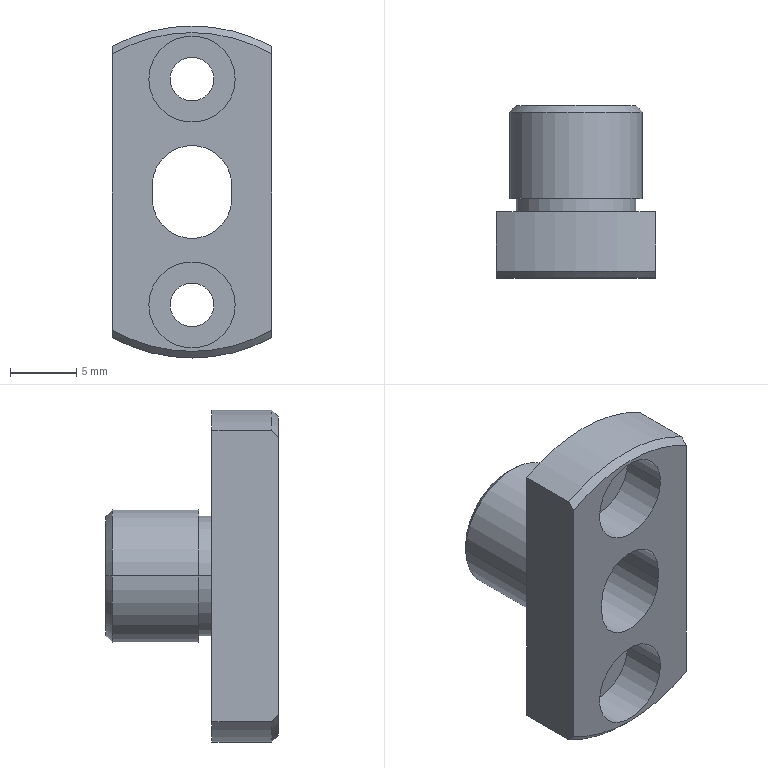Component | SolidWorks | F-JBEH10-P7-W6-L8-1 | 1 solid | 30 faces | box 12 x 13 x 25 mm | volume 1343 mm3 | cylinder 16 | plane 10 | cone 4 | commonest cylinder face diameters 3.3 x4 6.5 x4 9 x2 10 x2 25 x2 6 x2
STEP:
#1=COLOUR_RGB('',0.7922,0.8196,0.9333);
#2=FILL_AREA_STYLE_COLOUR('',#1);
#3=FILL_AREA_STYLE('',(#2));
#4=SURFACE_STYLE_FILL_AREA(#3);
#5=SURFACE_SIDE_STYLE('',(#4));
#6=SURFACE_STYLE_USAGE(.BOTH.,#5);
#7=PRESENTATION_STYLE_ASSIGNMENT((#6));
#8=CARTESIAN_POINT('',(-4.175,-1.116,4.536));
#9=VERTEX_POINT('',#8);
#10=CARTESIAN_POINT('',(-4.305,-1.116,4.536));
#11=VERTEX_POINT('',#10);
#12=CARTESIAN_POINT('',(-4.24,-1.116,4.536));
#13=DIRECTION('',(0.,1.,0.));
#14=DIRECTION('',(1.,0.,0.));
#15=AXIS2_PLACEMENT_3D('',#12,#13,#14);
#16=CIRCLE('',#15,0.06496);
#17=EDGE_CURVE('',#9,#11,#16,.T.);
#18=ORIENTED_EDGE('',*,*,#17,.T.);
#19=CARTESIAN_POINT('',(-4.305,-1.175,4.536));
#20=VERTEX_POINT('',#19);
#21=CARTESIAN_POINT('',(-4.305,-1.116,4.536));
#22=DIRECTION('',(0.,-1.,0.));
#23=VECTOR('',#22,39.37);
#24=LINE('',#21,#23);
#25=EDGE_CURVE('',#11,#20,#24,.T.);
#26=ORIENTED_EDGE('',*,*,#25,.T.);
#27=CARTESIAN_POINT('',(-4.175,-1.175,4.536));
#28=VERTEX_POINT('',#27);
#29=CARTESIAN_POINT('',(-4.24,-1.175,4.536));
#30=DIRECTION('',(0.,1.,0.));
#31=DIRECTION('',(1.,0.,0.));
#32=AXIS2_PLACEMENT_3D('',#29,#30,#31);
#33=CIRCLE('',#32,0.06496);
#34=EDGE_CURVE('',#28,#20,#33,.T.);
#35=ORIENTED_EDGE('',*,*,#34,.F.);
#36=CARTESIAN_POINT('',(-4.175,-1.116,4.536));
#37=DIRECTION('',(0.,-1.,0.));
#38=VECTOR('',#37,39.37);
#39=LINE('',#36,#38);
#40=EDGE_CURVE('',#9,#28,#39,.T.);
#41=ORIENTED_EDGE('',*,*,#40,.F.);
#42=EDGE_LOOP('',(#18,#26,#35,#41));
#43=FACE_OUTER_BOUND('',#42,.T.);
#44=CARTESIAN_POINT('',(-4.24,-1.116,4.536));
#45=DIRECTION('',(0.,-1.,0.));
#46=DIRECTION('',(1.,0.,0.));
#47=AXIS2_PLACEMENT_3D('',#44,#45,#46);
#48=CYLINDRICAL_SURFACE('',#47,0.06496);
#49=ADVANCED_FACE('',(#43),#48,.F.);
#50=CARTESIAN_POINT('',(-4.175,-1.116,5.206));
#51=VERTEX_POINT('',#50);
#52=CARTESIAN_POINT('',(-4.305,-1.116,5.206));
#53=VERTEX_POINT('',#52);
#54=CARTESIAN_POINT('',(-4.24,-1.116,5.206));
#55=DIRECTION('',(0.,1.,0.));
#56=DIRECTION('',(1.,0.,0.));
#57=AXIS2_PLACEMENT_3D('',#54,#55,#56);
#58=CIRCLE('',#57,0.06496);
#59=EDGE_CURVE('',#51,#53,#58,.T.);
#60=ORIENTED_EDGE('',*,*,#59,.T.);
#61=CARTESIAN_POINT('',(-4.305,-1.175,5.206));
#62=VERTEX_POINT('',#61);
#63=CARTESIAN_POINT('',(-4.305,-1.116,5.206));
#64=DIRECTION('',(0.,-1.,0.));
#65=VECTOR('',#64,39.37);
#66=LINE('',#63,#65);
#67=EDGE_CURVE('',#53,#62,#66,.T.);
#68=ORIENTED_EDGE('',*,*,#67,.T.);
#69=CARTESIAN_POINT('',(-4.175,-1.175,5.206));
#70=VERTEX_POINT('',#69);
#71=CARTESIAN_POINT('',(-4.24,-1.175,5.206));
#72=DIRECTION('',(0.,1.,0.));
#73=DIRECTION('',(1.,0.,0.));
#74=AXIS2_PLACEMENT_3D('',#71,#72,#73);
#75=CIRCLE('',#74,0.06496);
#76=EDGE_CURVE('',#70,#62,#75,.T.);
#77=ORIENTED_EDGE('',*,*,#76,.F.);
#78=CARTESIAN_POINT('',(-4.175,-1.116,5.206));
#79=DIRECTION('',(0.,-1.,0.));
#80=VECTOR('',#79,39.37);
#81=LINE('',#78,#80);
#82=EDGE_CURVE('',#51,#70,#81,.T.);
#83=ORIENTED_EDGE('',*,*,#82,.F.);
#84=EDGE_LOOP('',(#60,#68,#77,#83));
#85=FACE_OUTER_BOUND('',#84,.T.);
#86=CARTESIAN_POINT('',(-4.24,-1.116,5.206));
#87=DIRECTION('',(0.,-1.,0.));
#88=DIRECTION('',(1.,0.,0.));
#89=AXIS2_PLACEMENT_3D('',#86,#87,#88);
#90=CYLINDRICAL_SURFACE('',#89,0.06496);
#91=ADVANCED_FACE('',(#85),#90,.F.);
#92=CARTESIAN_POINT('',(-4.063,-1.076,4.871));
#93=VERTEX_POINT('',#92);
#94=CARTESIAN_POINT('',(-4.417,-1.076,4.871));
#95=VERTEX_POINT('',#94);
#96=CARTESIAN_POINT('',(-4.24,-1.076,4.871));
#97=DIRECTION('',(0.,-1.,0.));
#98=DIRECTION('',(1.,0.,0.));
#99=AXIS2_PLACEMENT_3D('',#96,#97,#98);
#100=CIRCLE('',#99,0.1772);
#101=EDGE_CURVE('',#93,#95,#100,.T.);
#102=ORIENTED_EDGE('',*,*,#101,.T.);
#103=CARTESIAN_POINT('',(-4.417,-1.116,4.871));
#104=VERTEX_POINT('',#103);
#105=CARTESIAN_POINT('',(-4.417,-0.8009,4.871));
#106=DIRECTION('',(0.,-1.,0.));
#107=VECTOR('',#106,39.37);
#108=LINE('',#105,#107);
#109=EDGE_CURVE('',#95,#104,#108,.T.);
#110=ORIENTED_EDGE('',*,*,#109,.T.);
#111=CARTESIAN_POINT('',(-4.063,-1.116,4.871));
#112=VERTEX_POINT('',#111);
#113=CARTESIAN_POINT('',(-4.24,-1.116,4.871));
#114=DIRECTION('',(0.,1.,0.));
#115=DIRECTION('',(1.,0.,0.));
#116=AXIS2_PLACEMENT_3D('',#113,#114,#115);
#117=CIRCLE('',#116,0.1772);
#118=EDGE_CURVE('',#104,#112,#117,.T.);
#119=ORIENTED_EDGE('',*,*,#118,.T.);
#120=CARTESIAN_POINT('',(-4.063,-0.8009,4.871));
#121=DIRECTION('',(0.,-1.,0.));
#122=VECTOR('',#121,39.37);
#123=LINE('',#120,#122);
#124=EDGE_CURVE('',#93,#112,#123,.T.);
#125=ORIENTED_EDGE('',*,*,#124,.F.);
#126=EDGE_LOOP('',(#102,#110,#119,#125));
#127=FACE_OUTER_BOUND('',#126,.T.);
#128=CARTESIAN_POINT('',(-4.24,-0.8009,4.871));
#129=DIRECTION('',(0.,-1.,0.));
#130=DIRECTION('',(1.,0.,0.));
#131=AXIS2_PLACEMENT_3D('',#128,#129,#130);
#132=CYLINDRICAL_SURFACE('',#131,0.1772);
#133=ADVANCED_FACE('',(#127),#132,.T.);
#134=CARTESIAN_POINT('',(-4.368,-1.175,4.536));
#135=VERTEX_POINT('',#134);
#136=CARTESIAN_POINT('',(-4.112,-1.175,4.536));
#137=VERTEX_POINT('',#136);
#138=CARTESIAN_POINT('',(-4.24,-1.175,4.536));
#139=DIRECTION('',(0.,-1.,0.));
#140=DIRECTION('',(1.,0.,0.));
#141=AXIS2_PLACEMENT_3D('',#138,#139,#140);
#142=CIRCLE('',#141,0.128);
#143=EDGE_CURVE('',#135,#137,#142,.T.);
#144=ORIENTED_EDGE('',*,*,#143,.F.);
#145=CARTESIAN_POINT('',(-4.368,-1.313,4.536));
#146=VERTEX_POINT('',#145);
#147=CARTESIAN_POINT('',(-4.368,-1.116,4.536));
#148=DIRECTION('',(0.,-1.,0.));
#149=VECTOR('',#148,39.37);
#150=LINE('',#147,#149);
#151=EDGE_CURVE('',#135,#146,#150,.T.);
#152=ORIENTED_EDGE('',*,*,#151,.T.);
#153=CARTESIAN_POINT('',(-4.112,-1.313,4.536));
#154=VERTEX_POINT('',#153);
#155=CARTESIAN_POINT('',(-4.24,-1.313,4.536));
#156=DIRECTION('',(0.,-1.,0.));
#157=DIRECTION('',(1.,0.,0.));
#158=AXIS2_PLACEMENT_3D('',#155,#156,#157);
#159=CIRCLE('',#158,0.128);
#160=EDGE_CURVE('',#146,#154,#159,.T.);
#161=ORIENTED_EDGE('',*,*,#160,.T.);
#162=CARTESIAN_POINT('',(-4.112,-1.116,4.536));
#163=DIRECTION('',(0.,-1.,0.));
#164=VECTOR('',#163,39.37);
#165=LINE('',#162,#164);
#166=EDGE_CURVE('',#137,#154,#165,.T.);
#167=ORIENTED_EDGE('',*,*,#166,.F.);
#168=EDGE_LOOP('',(#144,#152,#161,#167));
#169=FACE_OUTER_BOUND('',#168,.T.);
#170=CARTESIAN_POINT('',(-4.24,-1.116,4.536));
#171=DIRECTION('',(0.,-1.,0.));
#172=DIRECTION('',(1.,0.,0.));
#173=AXIS2_PLACEMENT_3D('',#170,#171,#172);
#174=CYLINDRICAL_SURFACE('',#173,0.128);
#175=ADVANCED_FACE('',(#169),#174,.F.);
#176=CARTESIAN_POINT('',(-4.368,-1.175,5.206));
#177=VERTEX_POINT('',#176);
#178=CARTESIAN_POINT('',(-4.112,-1.175,5.206));
#179=VERTEX_POINT('',#178);
#180=CARTESIAN_POINT('',(-4.24,-1.175,5.206));
#181=DIRECTION('',(0.,-1.,0.));
#182=DIRECTION('',(1.,0.,0.));
#183=AXIS2_PLACEMENT_3D('',#180,#181,#182);
#184=CIRCLE('',#183,0.128);
#185=EDGE_CURVE('',#177,#179,#184,.T.);
#186=ORIENTED_EDGE('',*,*,#185,.F.);
#187=CARTESIAN_POINT('',(-4.368,-1.313,5.206));
#188=VERTEX_POINT('',#187);
#189=CARTESIAN_POINT('',(-4.368,-1.116,5.206));
#190=DIRECTION('',(0.,-1.,0.));
#191=VECTOR('',#190,39.37);
#192=LINE('',#189,#191);
#193=EDGE_CURVE('',#177,#188,#192,.T.);
#194=ORIENTED_EDGE('',*,*,#193,.T.);
#195=CARTESIAN_POINT('',(-4.112,-1.313,5.206));
#196=VERTEX_POINT('',#195);
#197=CARTESIAN_POINT('',(-4.24,-1.313,5.206));
#198=DIRECTION('',(0.,-1.,0.));
#199=DIRECTION('',(1.,0.,0.));
#200=AXIS2_PLACEMENT_3D('',#197,#198,#199);
#201=CIRCLE('',#200,0.128);
#202=EDGE_CURVE('',#188,#196,#201,.T.);
#203=ORIENTED_EDGE('',*,*,#202,.T.);
#204=CARTESIAN_POINT('',(-4.112,-1.116,5.206));
#205=DIRECTION('',(0.,-1.,0.));
#206=VECTOR('',#205,39.37);
#207=LINE('',#204,#206);
#208=EDGE_CURVE('',#179,#196,#207,.T.);
#209=ORIENTED_EDGE('',*,*,#208,.F.);
#210=EDGE_LOOP('',(#186,#194,#203,#209));
#211=FACE_OUTER_BOUND('',#210,.T.);
#212=CARTESIAN_POINT('',(-4.24,-1.116,5.206));
#213=DIRECTION('',(0.,-1.,0.));
#214=DIRECTION('',(1.,0.,0.));
#215=AXIS2_PLACEMENT_3D('',#212,#213,#214);
#216=CYLINDRICAL_SURFACE('',#215,0.128);
#217=ADVANCED_FACE('',(#211),#216,.F.);
#218=CARTESIAN_POINT('',(-4.043,-0.8206,4.871));
#219=VERTEX_POINT('',#218);
#220=CARTESIAN_POINT('',(-4.437,-0.8206,4.871));
#221=VERTEX_POINT('',#220);
#222=CARTESIAN_POINT('',(-4.24,-0.8206,4.871));
#223=DIRECTION('',(0.,-1.,0.));
#224=DIRECTION('',(1.,0.,0.));
#225=AXIS2_PLACEMENT_3D('',#222,#223,#224);
#226=CIRCLE('',#225,0.1969);
#227=EDGE_CURVE('',#219,#221,#226,.T.);
#228=ORIENTED_EDGE('',*,*,#227,.T.);
#229=CARTESIAN_POINT('',(-4.437,-1.076,4.871));
#230=VERTEX_POINT('',#229);
#231=CARTESIAN_POINT('',(-4.437,-0.8009,4.871));
#232=DIRECTION('',(0.,-1.,0.));
#233=VECTOR('',#232,39.37);
#234=LINE('',#231,#233);
#235=EDGE_CURVE('',#221,#230,#234,.T.);
#236=ORIENTED_EDGE('',*,*,#235,.T.);
#237=CARTESIAN_POINT('',(-4.043,-1.076,4.871));
#238=VERTEX_POINT('',#237);
#239=CARTESIAN_POINT('',(-4.24,-1.076,4.871));
#240=DIRECTION('',(0.,1.,0.));
#241=DIRECTION('',(1.,0.,0.));
#242=AXIS2_PLACEMENT_3D('',#239,#240,#241);
#243=CIRCLE('',#242,0.1969);
#244=EDGE_CURVE('',#230,#238,#243,.T.);
#245=ORIENTED_EDGE('',*,*,#244,.T.);
#246=CARTESIAN_POINT('',(-4.043,-0.8009,4.871));
#247=DIRECTION('',(0.,-1.,0.));
#248=VECTOR('',#247,39.37);
#249=LINE('',#246,#248);
#250=EDGE_CURVE('',#219,#238,#249,.T.);
#251=ORIENTED_EDGE('',*,*,#250,.F.);
#252=EDGE_LOOP('',(#228,#236,#245,#251));
#253=FACE_OUTER_BOUND('',#252,.T.);
#254=CARTESIAN_POINT('',(-4.24,-0.8009,4.871));
#255=DIRECTION('',(0.,-1.,0.));
#256=DIRECTION('',(1.,0.,0.));
#257=AXIS2_PLACEMENT_3D('',#254,#255,#256);
#258=CYLINDRICAL_SURFACE('',#257,0.1969);
#259=ADVANCED_FACE('',(#253),#258,.T.);
#260=CARTESIAN_POINT('',(-4.063,-0.8009,4.871));
#261=VERTEX_POINT('',#260);
#262=CARTESIAN_POINT('',(-4.417,-0.8009,4.871));
#263=VERTEX_POINT('',#262);
#264=CARTESIAN_POINT('',(-4.24,-0.8009,4.871));
#265=DIRECTION('',(0.,-1.,0.));
#266=DIRECTION('',(1.,0.,0.));
#267=AXIS2_PLACEMENT_3D('',#264,#265,#266);
#268=CIRCLE('',#267,0.1772);
#269=EDGE_CURVE('',#261,#263,#268,.T.);
#270=ORIENTED_EDGE('',*,*,#269,.T.);
#271=CARTESIAN_POINT('',(-4.437,-0.8206,4.871));
#272=DIRECTION('',(-0.7071,-0.7071,0.));
#273=VECTOR('',#272,39.37);
#274=LINE('',#271,#273);
#275=EDGE_CURVE('',#263,#221,#274,.T.);
#276=ORIENTED_EDGE('',*,*,#275,.T.);
#277=ORIENTED_EDGE('',*,*,#227,.F.);
#278=CARTESIAN_POINT('',(-4.043,-0.8206,4.871));
#279=DIRECTION('',(0.7071,-0.7071,0.));
#280=VECTOR('',#279,39.37);
#281=LINE('',#278,#280);
#282=EDGE_CURVE('',#261,#219,#281,.T.);
#283=ORIENTED_EDGE('',*,*,#282,.F.);
#284=EDGE_LOOP('',(#270,#276,#277,#283));
#285=FACE_OUTER_BOUND('',#284,.T.);
#286=CARTESIAN_POINT('',(-4.24,-0.8206,4.871));
#287=DIRECTION('',(0.,-1.,0.));
#288=DIRECTION('',(1.,0.,0.));
#289=AXIS2_PLACEMENT_3D('',#286,#287,#288);
#290=CONICAL_SURFACE('',#289,0.1969,0.7854);
#291=ADVANCED_FACE('',(#285),#290,.T.);
#292=CARTESIAN_POINT('',(-4.003,-1.116,5.303));
#293=VERTEX_POINT('',#292);
#294=CARTESIAN_POINT('',(-4.476,-1.116,5.303));
#295=VERTEX_POINT('',#294);
#296=CARTESIAN_POINT('',(-4.24,-1.116,4.871));
#297=DIRECTION('',(0.,-1.,0.));
#298=DIRECTION('',(1.,0.,0.));
#299=AXIS2_PLACEMENT_3D('',#296,#297,#298);
#300=CIRCLE('',#299,0.4921);
#301=EDGE_CURVE('',#293,#295,#300,.T.);
#302=ORIENTED_EDGE('',*,*,#301,.F.);
#303=CARTESIAN_POINT('',(-4.003,-1.116,4.439));
#304=VERTEX_POINT('',#303);
#305=CARTESIAN_POINT('',(-4.003,-1.116,5.363));
#306=DIRECTION('',(0.,0.,1.));
#307=VECTOR('',#306,39.37);
#308=LINE('',#305,#307);
#309=EDGE_CURVE('',#304,#293,#308,.T.);
#310=ORIENTED_EDGE('',*,*,#309,.F.);
#311=CARTESIAN_POINT('',(-4.476,-1.116,4.439));
#312=VERTEX_POINT('',#311);
#313=CARTESIAN_POINT('',(-4.24,-1.116,4.871));
#314=DIRECTION('',(0.,-1.,0.));
#315=DIRECTION('',(1.,0.,0.));
#316=AXIS2_PLACEMENT_3D('',#313,#314,#315);
#317=CIRCLE('',#316,0.4921);
#318=EDGE_CURVE('',#312,#304,#317,.T.);
#319=ORIENTED_EDGE('',*,*,#318,.F.);
#320=CARTESIAN_POINT('',(-4.476,-1.116,5.363));
#321=DIRECTION('',(0.,0.,-1.));
#322=VECTOR('',#321,39.37);
#323=LINE('',#320,#322);
#324=EDGE_CURVE('',#295,#312,#323,.T.);
#325=ORIENTED_EDGE('',*,*,#324,.F.);
#326=EDGE_LOOP('',(#302,#310,#319,#325));
#327=FACE_OUTER_BOUND('',#326,.T.);
#328=ORIENTED_EDGE('',*,*,#17,.F.);
#329=CARTESIAN_POINT('',(-4.24,-1.116,4.536));
#330=DIRECTION('',(0.,1.,0.));
#331=DIRECTION('',(1.,0.,0.));
#332=AXIS2_PLACEMENT_3D('',#329,#330,#331);
#333=CIRCLE('',#332,0.06496);
#334=EDGE_CURVE('',#11,#9,#333,.T.);
#335=ORIENTED_EDGE('',*,*,#334,.F.);
#336=EDGE_LOOP('',(#328,#335));
#337=FACE_BOUND('',#336,.T.);
#338=ORIENTED_EDGE('',*,*,#59,.F.);
#339=CARTESIAN_POINT('',(-4.24,-1.116,5.206));
#340=DIRECTION('',(0.,1.,0.));
#341=DIRECTION('',(1.,0.,0.));
#342=AXIS2_PLACEMENT_3D('',#339,#340,#341);
#343=CIRCLE('',#342,0.06496);
#344=EDGE_CURVE('',#53,#51,#343,.T.);
#345=ORIENTED_EDGE('',*,*,#344,.F.);
#346=EDGE_LOOP('',(#338,#345));
#347=FACE_BOUND('',#346,.T.);
#348=CARTESIAN_POINT('',(-4.24,-1.116,4.871));
#349=DIRECTION('',(0.,1.,0.));
#350=DIRECTION('',(1.,0.,0.));
#351=AXIS2_PLACEMENT_3D('',#348,#349,#350);
#352=CIRCLE('',#351,0.1772);
#353=EDGE_CURVE('',#112,#104,#352,.T.);
#354=ORIENTED_EDGE('',*,*,#353,.F.);
#355=ORIENTED_EDGE('',*,*,#118,.F.);
#356=EDGE_LOOP('',(#354,#355));
#357=FACE_BOUND('',#356,.T.);
#358=CARTESIAN_POINT('',(-4.24,-1.116,5.363));
#359=DIRECTION('',(0.,-1.,0.));
#360=DIRECTION('',(1.,0.,0.));
#361=AXIS2_PLACEMENT_3D('',#358,#359,#360);
#362=PLANE('',#361);
#363=ADVANCED_FACE('',(#327,#337,#347,#357),#362,.F.);
#364=CARTESIAN_POINT('',(-4.476,-1.313,4.462));
#365=VERTEX_POINT('',#364);
#366=CARTESIAN_POINT('',(-4.476,-1.293,4.439));
#367=VERTEX_POINT('',#366);
#368=CARTESIAN_POINT('',(-4.476,-1.313,4.462));
#369=CARTESIAN_POINT('',(-4.476,-1.306,4.454));
#370=CARTESIAN_POINT('',(-4.476,-1.3,4.447));
#371=CARTESIAN_POINT('',(-4.476,-1.293,4.439));
#372=B_SPLINE_CURVE_WITH_KNOTS('',3,(#368,#369,#370,#371),.UNSPECIFIED.,.F.,.F.,(4,4),(0.,0.0007609),.UNSPECIFIED.);
#373=EDGE_CURVE('',#365,#367,#372,.T.);
#374=ORIENTED_EDGE('',*,*,#373,.F.);
#375=CARTESIAN_POINT('',(-4.476,-1.313,5.28));
#376=VERTEX_POINT('',#375);
#377=CARTESIAN_POINT('',(-4.476,-1.313,5.363));
#378=DIRECTION('',(0.,0.,1.));
#379=VECTOR('',#378,39.37);
#380=LINE('',#377,#379);
#381=EDGE_CURVE('',#365,#376,#380,.T.);
#382=ORIENTED_EDGE('',*,*,#381,.T.);
#383=CARTESIAN_POINT('',(-4.476,-1.293,5.303));
#384=VERTEX_POINT('',#383);
#385=CARTESIAN_POINT('',(-4.476,-1.293,5.303));
#386=CARTESIAN_POINT('',(-4.476,-1.3,5.295));
#387=CARTESIAN_POINT('',(-4.476,-1.306,5.288));
#388=CARTESIAN_POINT('',(-4.476,-1.313,5.28));
#389=B_SPLINE_CURVE_WITH_KNOTS('',3,(#385,#386,#387,#388),.UNSPECIFIED.,.F.,.F.,(4,4),(0.,0.0007609),.UNSPECIFIED.);
#390=EDGE_CURVE('',#384,#376,#389,.T.);
#391=ORIENTED_EDGE('',*,*,#390,.F.);
#392=CARTESIAN_POINT('',(-4.476,-1.116,5.303));
#393=DIRECTION('',(0.,1.,0.));
#394=VECTOR('',#393,39.37);
#395=LINE('',#392,#394);
#396=EDGE_CURVE('',#384,#295,#395,.T.);
#397=ORIENTED_EDGE('',*,*,#396,.T.);
#398=ORIENTED_EDGE('',*,*,#324,.T.);
#399=CARTESIAN_POINT('',(-4.476,-1.116,4.439));
#400=DIRECTION('',(0.,-1.,0.));
#401=VECTOR('',#400,39.37);
#402=LINE('',#399,#401);
#403=EDGE_CURVE('',#312,#367,#402,.T.);
#404=ORIENTED_EDGE('',*,*,#403,.T.);
#405=EDGE_LOOP('',(#374,#382,#391,#397,#398,#404));
#406=FACE_OUTER_BOUND('',#405,.T.);
#407=CARTESIAN_POINT('',(-4.476,-1.116,5.363));
#408=DIRECTION('',(-1.,0.,0.));
#409=DIRECTION('',(0.,-1.,0.));
#410=AXIS2_PLACEMENT_3D('',#407,#408,#409);
#411=PLANE('',#410);
#412=ADVANCED_FACE('',(#406),#411,.T.);
#413=ORIENTED_EDGE('',*,*,#396,.F.);
#414=CARTESIAN_POINT('',(-4.003,-1.293,5.303));
#415=VERTEX_POINT('',#414);
#416=CARTESIAN_POINT('',(-4.24,-1.293,4.871));
#417=DIRECTION('',(0.,1.,0.));
#418=DIRECTION('',(1.,0.,-0.));
#419=AXIS2_PLACEMENT_3D('',#416,#417,#418);
#420=CIRCLE('',#419,0.4921);
#421=EDGE_CURVE('',#384,#415,#420,.T.);
#422=ORIENTED_EDGE('',*,*,#421,.T.);
#423=CARTESIAN_POINT('',(-4.003,-0.8009,5.303));
#424=DIRECTION('',(0.,1.,0.));
#425=VECTOR('',#424,39.37);
#426=LINE('',#423,#425);
#427=EDGE_CURVE('',#415,#293,#426,.T.);
#428=ORIENTED_EDGE('',*,*,#427,.T.);
#429=ORIENTED_EDGE('',*,*,#301,.T.);
#430=EDGE_LOOP('',(#413,#422,#428,#429));
#431=FACE_OUTER_BOUND('',#430,.T.);
#432=CARTESIAN_POINT('',(-4.24,-0.8009,4.871));
#433=DIRECTION('',(0.,-1.,0.));
#434=DIRECTION('',(1.,0.,0.));
#435=AXIS2_PLACEMENT_3D('',#432,#433,#434);
#436=CYLINDRICAL_SURFACE('',#435,0.4921);
#437=ADVANCED_FACE('',(#431),#436,.T.);
#438=CARTESIAN_POINT('',(-4.003,-1.313,5.28));
#439=VERTEX_POINT('',#438);
#440=CARTESIAN_POINT('',(-4.003,-1.293,5.303));
#441=CARTESIAN_POINT('',(-4.003,-1.3,5.295));
#442=CARTESIAN_POINT('',(-4.003,-1.306,5.288));
#443=CARTESIAN_POINT('',(-4.003,-1.313,5.28));
#444=B_SPLINE_CURVE_WITH_KNOTS('',3,(#440,#441,#442,#443),.UNSPECIFIED.,.F.,.F.,(4,4),(0.,0.0007609),.UNSPECIFIED.);
#445=EDGE_CURVE('',#415,#439,#444,.T.);
#446=ORIENTED_EDGE('',*,*,#445,.T.);
#447=CARTESIAN_POINT('',(-4.003,-1.313,4.462));
#448=VERTEX_POINT('',#447);
#449=CARTESIAN_POINT('',(-4.003,-1.313,4.379));
#450=DIRECTION('',(0.,0.,-1.));
#451=VECTOR('',#450,39.37);
#452=LINE('',#449,#451);
#453=EDGE_CURVE('',#439,#448,#452,.T.);
#454=ORIENTED_EDGE('',*,*,#453,.T.);
#455=CARTESIAN_POINT('',(-4.003,-1.293,4.439));
#456=VERTEX_POINT('',#455);
#457=CARTESIAN_POINT('',(-4.003,-1.293,4.439));
#458=CARTESIAN_POINT('',(-4.003,-1.3,4.447));
#459=CARTESIAN_POINT('',(-4.003,-1.306,4.454));
#460=CARTESIAN_POINT('',(-4.003,-1.313,4.462));
#461=B_SPLINE_CURVE_WITH_KNOTS('',3,(#457,#458,#459,#460),.UNSPECIFIED.,.F.,.F.,(4,4),(0.,0.0007609),.UNSPECIFIED.);
#462=EDGE_CURVE('',#456,#448,#461,.T.);
#463=ORIENTED_EDGE('',*,*,#462,.F.);
#464=CARTESIAN_POINT('',(-4.003,-1.116,4.439));
#465=DIRECTION('',(0.,1.,0.));
#466=VECTOR('',#465,39.37);
#467=LINE('',#464,#466);
#468=EDGE_CURVE('',#456,#304,#467,.T.);
#469=ORIENTED_EDGE('',*,*,#468,.T.);
#470=ORIENTED_EDGE('',*,*,#309,.T.);
#471=ORIENTED_EDGE('',*,*,#427,.F.);
#472=EDGE_LOOP('',(#446,#454,#463,#469,#470,#471));
#473=FACE_OUTER_BOUND('',#472,.T.);
#474=CARTESIAN_POINT('',(-4.003,-1.116,4.379));
#475=DIRECTION('',(1.,0.,0.));
#476=DIRECTION('',(0.,1.,0.));
#477=AXIS2_PLACEMENT_3D('',#474,#475,#476);
#478=PLANE('',#477);
#479=ADVANCED_FACE('',(#473),#478,.T.);
#480=ORIENTED_EDGE('',*,*,#403,.F.);
#481=ORIENTED_EDGE('',*,*,#318,.T.);
#482=ORIENTED_EDGE('',*,*,#468,.F.);
#483=CARTESIAN_POINT('',(-4.24,-1.293,4.871));
#484=DIRECTION('',(0.,1.,0.));
#485=DIRECTION('',(1.,0.,0.));
#486=AXIS2_PLACEMENT_3D('',#483,#484,#485);
#487=CIRCLE('',#486,0.4921);
#488=EDGE_CURVE('',#456,#367,#487,.T.);
#489=ORIENTED_EDGE('',*,*,#488,.T.);
#490=EDGE_LOOP('',(#480,#481,#482,#489));
#491=FACE_OUTER_BOUND('',#490,.T.);
#492=CARTESIAN_POINT('',(-4.24,-0.8009,4.871));
#493=DIRECTION('',(0.,-1.,0.));
#494=DIRECTION('',(1.,0.,0.));
#495=AXIS2_PLACEMENT_3D('',#492,#493,#494);
#496=CYLINDRICAL_SURFACE('',#495,0.4921);
#497=ADVANCED_FACE('',(#491),#496,.T.);
#498=ORIENTED_EDGE('',*,*,#25,.F.);
#499=ORIENTED_EDGE('',*,*,#334,.T.);
#500=ORIENTED_EDGE('',*,*,#40,.T.);
#501=CARTESIAN_POINT('',(-4.24,-1.175,4.536));
#502=DIRECTION('',(0.,1.,0.));
#503=DIRECTION('',(1.,0.,0.));
#504=AXIS2_PLACEMENT_3D('',#501,#502,#503);
#505=CIRCLE('',#504,0.06496);
#506=EDGE_CURVE('',#20,#28,#505,.T.);
#507=ORIENTED_EDGE('',*,*,#506,.F.);
#508=EDGE_LOOP('',(#498,#499,#500,#507));
#509=FACE_OUTER_BOUND('',#508,.T.);
#510=CARTESIAN_POINT('',(-4.24,-1.116,4.536));
#511=DIRECTION('',(0.,-1.,0.));
#512=DIRECTION('',(1.,0.,0.));
#513=AXIS2_PLACEMENT_3D('',#510,#511,#512);
#514=CYLINDRICAL_SURFACE('',#513,0.06496);
#515=ADVANCED_FACE('',(#509),#514,.F.);
#516=ORIENTED_EDGE('',*,*,#67,.F.);
#517=ORIENTED_EDGE('',*,*,#344,.T.);
#518=ORIENTED_EDGE('',*,*,#82,.T.);
#519=CARTESIAN_POINT('',(-4.24,-1.175,5.206));
#520=DIRECTION('',(0.,1.,0.));
#521=DIRECTION('',(1.,0.,0.));
#522=AXIS2_PLACEMENT_3D('',#519,#520,#521);
#523=CIRCLE('',#522,0.06496);
#524=EDGE_CURVE('',#62,#70,#523,.T.);
#525=ORIENTED_EDGE('',*,*,#524,.F.);
#526=EDGE_LOOP('',(#516,#517,#518,#525));
#527=FACE_OUTER_BOUND('',#526,.T.);
#528=CARTESIAN_POINT('',(-4.24,-1.116,5.206));
#529=DIRECTION('',(0.,-1.,0.));
#530=DIRECTION('',(1.,0.,0.));
#531=AXIS2_PLACEMENT_3D('',#528,#529,#530);
#532=CYLINDRICAL_SURFACE('',#531,0.06496);
#533=ADVANCED_FACE('',(#527),#532,.F.);
#534=ORIENTED_EDGE('',*,*,#109,.F.);
#535=CARTESIAN_POINT('',(-4.24,-1.076,4.871));
#536=DIRECTION('',(0.,-1.,0.));
#537=DIRECTION('',(1.,0.,0.));
#538=AXIS2_PLACEMENT_3D('',#535,#536,#537);
#539=CIRCLE('',#538,0.1772);
#540=EDGE_CURVE('',#95,#93,#539,.T.);
#541=ORIENTED_EDGE('',*,*,#540,.T.);
#542=ORIENTED_EDGE('',*,*,#124,.T.);
#543=ORIENTED_EDGE('',*,*,#353,.T.);
#544=EDGE_LOOP('',(#534,#541,#542,#543));
#545=FACE_OUTER_BOUND('',#544,.T.);
#546=CARTESIAN_POINT('',(-4.24,-0.8009,4.871));
#547=DIRECTION('',(0.,-1.,0.));
#548=DIRECTION('',(1.,0.,0.));
#549=AXIS2_PLACEMENT_3D('',#546,#547,#548);
#550=CYLINDRICAL_SURFACE('',#549,0.1772);
#551=ADVANCED_FACE('',(#545),#550,.T.);
#552=CARTESIAN_POINT('',(-4.122,-1.313,4.891));
#553=VERTEX_POINT('',#552);
#554=CARTESIAN_POINT('',(-4.358,-1.313,4.891));
#555=VERTEX_POINT('',#554);
#556=CARTESIAN_POINT('',(-4.24,-1.313,4.891));
#557=DIRECTION('',(0.,-1.,0.));
#558=DIRECTION('',(-1.,0.,0.));
#559=AXIS2_PLACEMENT_3D('',#556,#557,#558);
#560=CIRCLE('',#559,0.1181);
#561=EDGE_CURVE('',#553,#555,#560,.T.);
#562=ORIENTED_EDGE('',*,*,#561,.F.);
#563=CARTESIAN_POINT('',(-4.122,-1.313,4.851));
#564=VERTEX_POINT('',#563);
#565=CARTESIAN_POINT('',(-4.122,-1.313,4.851));
#566=DIRECTION('',(0.,0.,-1.));
#567=VECTOR('',#566,39.37);
#568=LINE('',#565,#567);
#569=EDGE_CURVE('',#553,#564,#568,.T.);
#570=ORIENTED_EDGE('',*,*,#569,.T.);
#571=CARTESIAN_POINT('',(-4.358,-1.313,4.851));
#572=VERTEX_POINT('',#571);
#573=CARTESIAN_POINT('',(-4.24,-1.313,4.851));
#574=DIRECTION('',(0.,-1.,0.));
#575=DIRECTION('',(-1.,0.,0.));
#576=AXIS2_PLACEMENT_3D('',#573,#574,#575);
#577=CIRCLE('',#576,0.1181);
#578=EDGE_CURVE('',#572,#564,#577,.T.);
#579=ORIENTED_EDGE('',*,*,#578,.F.);
#580=CARTESIAN_POINT('',(-4.358,-1.313,4.891));
#581=DIRECTION('',(0.,0.,1.));
#582=VECTOR('',#581,39.37);
#583=LINE('',#580,#582);
#584=EDGE_CURVE('',#572,#555,#583,.T.);
#585=ORIENTED_EDGE('',*,*,#584,.T.);
#586=EDGE_LOOP('',(#562,#570,#579,#585));
#587=FACE_BOUND('',#586,.T.);
#588=CARTESIAN_POINT('',(-4.24,-1.313,4.536));
#589=DIRECTION('',(0.,-1.,0.));
#590=DIRECTION('',(1.,0.,0.));
#591=AXIS2_PLACEMENT_3D('',#588,#589,#590);
#592=CIRCLE('',#591,0.128);
#593=EDGE_CURVE('',#154,#146,#592,.T.);
#594=ORIENTED_EDGE('',*,*,#593,.F.);
#595=ORIENTED_EDGE('',*,*,#160,.F.);
#596=EDGE_LOOP('',(#594,#595));
#597=FACE_BOUND('',#596,.T.);
#598=CARTESIAN_POINT('',(-4.24,-1.313,5.206));
#599=DIRECTION('',(0.,-1.,0.));
#600=DIRECTION('',(1.,0.,0.));
#601=AXIS2_PLACEMENT_3D('',#598,#599,#600);
#602=CIRCLE('',#601,0.128);
#603=EDGE_CURVE('',#196,#188,#602,.T.);
#604=ORIENTED_EDGE('',*,*,#603,.F.);
#605=ORIENTED_EDGE('',*,*,#202,.F.);
#606=EDGE_LOOP('',(#604,#605));
#607=FACE_BOUND('',#606,.T.);
#608=ORIENTED_EDGE('',*,*,#381,.F.);
#609=CARTESIAN_POINT('',(-4.24,-1.313,4.871));
#610=DIRECTION('',(0.,1.,0.));
#611=DIRECTION('',(-1.,0.,0.));
#612=AXIS2_PLACEMENT_3D('',#609,#610,#611);
#613=CIRCLE('',#612,0.4724);
#614=EDGE_CURVE('',#448,#365,#613,.T.);
#615=ORIENTED_EDGE('',*,*,#614,.F.);
#616=ORIENTED_EDGE('',*,*,#453,.F.);
#617=CARTESIAN_POINT('',(-4.24,-1.313,4.871));
#618=DIRECTION('',(0.,1.,0.));
#619=DIRECTION('',(-1.,0.,0.));
#620=AXIS2_PLACEMENT_3D('',#617,#618,#619);
#621=CIRCLE('',#620,0.4724);
#622=EDGE_CURVE('',#376,#439,#621,.T.);
#623=ORIENTED_EDGE('',*,*,#622,.F.);
#624=EDGE_LOOP('',(#608,#615,#616,#623));
#625=FACE_OUTER_BOUND('',#624,.T.);
#626=CARTESIAN_POINT('',(-4.24,-1.313,4.871));
#627=DIRECTION('',(0.,1.,0.));
#628=DIRECTION('',(-1.,0.,0.));
#629=AXIS2_PLACEMENT_3D('',#626,#627,#628);
#630=PLANE('',#629);
#631=ADVANCED_FACE('',(#587,#597,#607,#625),#630,.F.);
#632=ORIENTED_EDGE('',*,*,#390,.T.);
#633=ORIENTED_EDGE('',*,*,#622,.T.);
#634=ORIENTED_EDGE('',*,*,#445,.F.);
#635=ORIENTED_EDGE('',*,*,#421,.F.);
#636=EDGE_LOOP('',(#632,#633,#634,#635));
#637=FACE_OUTER_BOUND('',#636,.T.);
#638=CARTESIAN_POINT('',(-4.24,-1.293,4.871));
#639=DIRECTION('',(0.,1.,0.));
#640=DIRECTION('',(-1.,0.,0.));
#641=AXIS2_PLACEMENT_3D('',#638,#639,#640);
#642=CONICAL_SURFACE('',#641,0.4921,0.7854);
#643=ADVANCED_FACE('',(#637),#642,.T.);
#644=ORIENTED_EDGE('',*,*,#462,.T.);
#645=ORIENTED_EDGE('',*,*,#614,.T.);
#646=ORIENTED_EDGE('',*,*,#373,.T.);
#647=ORIENTED_EDGE('',*,*,#488,.F.);
#648=EDGE_LOOP('',(#644,#645,#646,#647));
#649=FACE_OUTER_BOUND('',#648,.T.);
#650=CARTESIAN_POINT('',(-4.24,-1.293,4.871));
#651=DIRECTION('',(0.,1.,0.));
#652=DIRECTION('',(-1.,0.,0.));
#653=AXIS2_PLACEMENT_3D('',#650,#651,#652);
#654=CONICAL_SURFACE('',#653,0.4921,0.7854);
#655=ADVANCED_FACE('',(#649),#654,.T.);
#656=CARTESIAN_POINT('',(-4.24,-1.175,4.536));
#657=DIRECTION('',(0.,-1.,0.));
#658=DIRECTION('',(1.,0.,0.));
#659=AXIS2_PLACEMENT_3D('',#656,#657,#658);
#660=CIRCLE('',#659,0.128);
#661=EDGE_CURVE('',#137,#135,#660,.T.);
#662=ORIENTED_EDGE('',*,*,#661,.T.);
#663=ORIENTED_EDGE('',*,*,#143,.T.);
#664=EDGE_LOOP('',(#662,#663));
#665=FACE_OUTER_BOUND('',#664,.T.);
#666=ORIENTED_EDGE('',*,*,#34,.T.);
#667=ORIENTED_EDGE('',*,*,#506,.T.);
#668=EDGE_LOOP('',(#666,#667));
#669=FACE_BOUND('',#668,.T.);
#670=CARTESIAN_POINT('',(-4.24,-1.175,4.664));
#671=DIRECTION('',(0.,-1.,0.));
#672=DIRECTION('',(1.,0.,0.));
#673=AXIS2_PLACEMENT_3D('',#670,#671,#672);
#674=PLANE('',#673);
#675=ADVANCED_FACE('',(#665,#669),#674,.T.);
#676=CARTESIAN_POINT('',(-4.24,-1.175,5.206));
#677=DIRECTION('',(0.,-1.,0.));
#678=DIRECTION('',(1.,0.,0.));
#679=AXIS2_PLACEMENT_3D('',#676,#677,#678);
#680=CIRCLE('',#679,0.128);
#681=EDGE_CURVE('',#179,#177,#680,.T.);
#682=ORIENTED_EDGE('',*,*,#681,.T.);
#683=ORIENTED_EDGE('',*,*,#185,.T.);
#684=EDGE_LOOP('',(#682,#683));
#685=FACE_OUTER_BOUND('',#684,.T.);
#686=ORIENTED_EDGE('',*,*,#76,.T.);
#687=ORIENTED_EDGE('',*,*,#524,.T.);
#688=EDGE_LOOP('',(#686,#687));
#689=FACE_BOUND('',#688,.T.);
#690=CARTESIAN_POINT('',(-4.24,-1.175,5.333));
#691=DIRECTION('',(0.,-1.,0.));
#692=DIRECTION('',(1.,0.,0.));
#693=AXIS2_PLACEMENT_3D('',#690,#691,#692);
#694=PLANE('',#693);
#695=ADVANCED_FACE('',(#685,#689),#694,.T.);
#696=ORIENTED_EDGE('',*,*,#101,.F.);
#697=ORIENTED_EDGE('',*,*,#540,.F.);
#698=EDGE_LOOP('',(#696,#697));
#699=FACE_BOUND('',#698,.T.);
#700=CARTESIAN_POINT('',(-4.24,-1.076,4.871));
#701=DIRECTION('',(0.,1.,0.));
#702=DIRECTION('',(1.,0.,0.));
#703=AXIS2_PLACEMENT_3D('',#700,#701,#702);
#704=CIRCLE('',#703,0.1969);
#705=EDGE_CURVE('',#238,#230,#704,.T.);
#706=ORIENTED_EDGE('',*,*,#705,.F.);
#707=ORIENTED_EDGE('',*,*,#244,.F.);
#708=EDGE_LOOP('',(#706,#707));
#709=FACE_OUTER_BOUND('',#708,.T.);
#710=CARTESIAN_POINT('',(-4.24,-1.076,5.048));
#711=DIRECTION('',(0.,1.,0.));
#712=DIRECTION('',(-1.,0.,0.));
#713=AXIS2_PLACEMENT_3D('',#710,#711,#712);
#714=PLANE('',#713);
#715=ADVANCED_FACE('',(#699,#709),#714,.F.);
#716=CARTESIAN_POINT('',(-4.358,-0.8009,4.891));
#717=VERTEX_POINT('',#716);
#718=CARTESIAN_POINT('',(-4.358,-0.8009,4.891));
#719=DIRECTION('',(0.,-1.,0.));
#720=VECTOR('',#719,39.37);
#721=LINE('',#718,#720);
#722=EDGE_CURVE('',#717,#555,#721,.T.);
#723=ORIENTED_EDGE('',*,*,#722,.F.);
#724=CARTESIAN_POINT('',(-4.122,-0.8009,4.891));
#725=VERTEX_POINT('',#724);
#726=CARTESIAN_POINT('',(-4.24,-0.8009,4.891));
#727=DIRECTION('',(0.,-1.,0.));
#728=DIRECTION('',(-1.,0.,0.));
#729=AXIS2_PLACEMENT_3D('',#726,#727,#728);
#730=CIRCLE('',#729,0.1181);
#731=EDGE_CURVE('',#725,#717,#730,.T.);
#732=ORIENTED_EDGE('',*,*,#731,.F.);
#733=CARTESIAN_POINT('',(-4.122,-0.8009,4.891));
#734=DIRECTION('',(0.,1.,0.));
#735=VECTOR('',#734,39.37);
#736=LINE('',#733,#735);
#737=EDGE_CURVE('',#553,#725,#736,.T.);
#738=ORIENTED_EDGE('',*,*,#737,.F.);
#739=ORIENTED_EDGE('',*,*,#561,.T.);
#740=EDGE_LOOP('',(#723,#732,#738,#739));
#741=FACE_OUTER_BOUND('',#740,.T.);
#742=CARTESIAN_POINT('',(-4.24,-0.8009,4.891));
#743=DIRECTION('',(0.,1.,0.));
#744=DIRECTION('',(-1.,0.,0.));
#745=AXIS2_PLACEMENT_3D('',#742,#743,#744);
#746=CYLINDRICAL_SURFACE('',#745,0.1181);
#747=ADVANCED_FACE('',(#741),#746,.F.);
#748=CARTESIAN_POINT('',(-4.122,-0.8009,4.851));
#749=VERTEX_POINT('',#748);
#750=CARTESIAN_POINT('',(-4.122,-0.8009,4.851));
#751=DIRECTION('',(0.,-1.,0.));
#752=VECTOR('',#751,39.37);
#753=LINE('',#750,#752);
#754=EDGE_CURVE('',#749,#564,#753,.T.);
#755=ORIENTED_EDGE('',*,*,#754,.F.);
#756=CARTESIAN_POINT('',(-4.358,-0.8009,4.851));
#757=VERTEX_POINT('',#756);
#758=CARTESIAN_POINT('',(-4.24,-0.8009,4.851));
#759=DIRECTION('',(0.,-1.,0.));
#760=DIRECTION('',(-1.,0.,0.));
#761=AXIS2_PLACEMENT_3D('',#758,#759,#760);
#762=CIRCLE('',#761,0.1181);
#763=EDGE_CURVE('',#757,#749,#762,.T.);
#764=ORIENTED_EDGE('',*,*,#763,.F.);
#765=CARTESIAN_POINT('',(-4.358,-0.8009,4.851));
#766=DIRECTION('',(0.,1.,0.));
#767=VECTOR('',#766,39.37);
#768=LINE('',#765,#767);
#769=EDGE_CURVE('',#572,#757,#768,.T.);
#770=ORIENTED_EDGE('',*,*,#769,.F.);
#771=ORIENTED_EDGE('',*,*,#578,.T.);
#772=EDGE_LOOP('',(#755,#764,#770,#771));
#773=FACE_OUTER_BOUND('',#772,.T.);
#774=CARTESIAN_POINT('',(-4.24,-0.8009,4.851));
#775=DIRECTION('',(0.,1.,0.));
#776=DIRECTION('',(-1.,0.,0.));
#777=AXIS2_PLACEMENT_3D('',#774,#775,#776);
#778=CYLINDRICAL_SURFACE('',#777,0.1181);
#779=ADVANCED_FACE('',(#773),#778,.F.);
#780=ORIENTED_EDGE('',*,*,#151,.F.);
#781=ORIENTED_EDGE('',*,*,#661,.F.);
#782=ORIENTED_EDGE('',*,*,#166,.T.);
#783=ORIENTED_EDGE('',*,*,#593,.T.);
#784=EDGE_LOOP('',(#780,#781,#782,#783));
#785=FACE_OUTER_BOUND('',#784,.T.);
#786=CARTESIAN_POINT('',(-4.24,-1.116,4.536));
#787=DIRECTION('',(0.,-1.,0.));
#788=DIRECTION('',(1.,0.,0.));
#789=AXIS2_PLACEMENT_3D('',#786,#787,#788);
#790=CYLINDRICAL_SURFACE('',#789,0.128);
#791=ADVANCED_FACE('',(#785),#790,.F.);
#792=ORIENTED_EDGE('',*,*,#193,.F.);
#793=ORIENTED_EDGE('',*,*,#681,.F.);
#794=ORIENTED_EDGE('',*,*,#208,.T.);
#795=ORIENTED_EDGE('',*,*,#603,.T.);
#796=EDGE_LOOP('',(#792,#793,#794,#795));
#797=FACE_OUTER_BOUND('',#796,.T.);
#798=CARTESIAN_POINT('',(-4.24,-1.116,5.206));
#799=DIRECTION('',(0.,-1.,0.));
#800=DIRECTION('',(1.,0.,0.));
#801=AXIS2_PLACEMENT_3D('',#798,#799,#800);
#802=CYLINDRICAL_SURFACE('',#801,0.128);
#803=ADVANCED_FACE('',(#797),#802,.F.);
#804=ORIENTED_EDGE('',*,*,#235,.F.);
#805=CARTESIAN_POINT('',(-4.24,-0.8206,4.871));
#806=DIRECTION('',(0.,-1.,0.));
#807=DIRECTION('',(1.,0.,0.));
#808=AXIS2_PLACEMENT_3D('',#805,#806,#807);
#809=CIRCLE('',#808,0.1969);
#810=EDGE_CURVE('',#221,#219,#809,.T.);
#811=ORIENTED_EDGE('',*,*,#810,.T.);
#812=ORIENTED_EDGE('',*,*,#250,.T.);
#813=ORIENTED_EDGE('',*,*,#705,.T.);
#814=EDGE_LOOP('',(#804,#811,#812,#813));
#815=FACE_OUTER_BOUND('',#814,.T.);
#816=CARTESIAN_POINT('',(-4.24,-0.8009,4.871));
#817=DIRECTION('',(0.,-1.,0.));
#818=DIRECTION('',(1.,0.,0.));
#819=AXIS2_PLACEMENT_3D('',#816,#817,#818);
#820=CYLINDRICAL_SURFACE('',#819,0.1969);
#821=ADVANCED_FACE('',(#815),#820,.T.);
#822=ORIENTED_EDGE('',*,*,#769,.T.);
#823=CARTESIAN_POINT('',(-4.358,-0.8009,4.891));
#824=DIRECTION('',(0.,0.,-1.));
#825=VECTOR('',#824,39.37);
#826=LINE('',#823,#825);
#827=EDGE_CURVE('',#717,#757,#826,.T.);
#828=ORIENTED_EDGE('',*,*,#827,.F.);
#829=ORIENTED_EDGE('',*,*,#722,.T.);
#830=ORIENTED_EDGE('',*,*,#584,.F.);
#831=EDGE_LOOP('',(#822,#828,#829,#830));
#832=FACE_OUTER_BOUND('',#831,.T.);
#833=CARTESIAN_POINT('',(-4.358,-0.8009,4.891));
#834=DIRECTION('',(-1.,0.,0.));
#835=DIRECTION('',(0.,-1.,0.));
#836=AXIS2_PLACEMENT_3D('',#833,#834,#835);
#837=PLANE('',#836);
#838=ADVANCED_FACE('',(#832),#837,.F.);
#839=ORIENTED_EDGE('',*,*,#269,.F.);
#840=CARTESIAN_POINT('',(-4.24,-0.8009,4.871));
#841=DIRECTION('',(0.,-1.,0.));
#842=DIRECTION('',(1.,0.,0.));
#843=AXIS2_PLACEMENT_3D('',#840,#841,#842);
#844=CIRCLE('',#843,0.1772);
#845=EDGE_CURVE('',#263,#261,#844,.T.);
#846=ORIENTED_EDGE('',*,*,#845,.F.);
#847=EDGE_LOOP('',(#839,#846));
#848=FACE_OUTER_BOUND('',#847,.T.);
#849=ORIENTED_EDGE('',*,*,#731,.T.);
#850=ORIENTED_EDGE('',*,*,#827,.T.);
#851=ORIENTED_EDGE('',*,*,#763,.T.);
#852=CARTESIAN_POINT('',(-4.122,-0.8009,5.048));
#853=DIRECTION('',(0.,0.,-1.));
#854=VECTOR('',#853,39.37);
#855=LINE('',#852,#854);
#856=EDGE_CURVE('',#725,#749,#855,.T.);
#857=ORIENTED_EDGE('',*,*,#856,.F.);
#858=EDGE_LOOP('',(#849,#850,#851,#857));
#859=FACE_BOUND('',#858,.T.);
#860=CARTESIAN_POINT('',(-4.24,-0.8009,5.048));
#861=DIRECTION('',(0.,-1.,0.));
#862=DIRECTION('',(1.,0.,0.));
#863=AXIS2_PLACEMENT_3D('',#860,#861,#862);
#864=PLANE('',#863);
#865=ADVANCED_FACE('',(#848,#859),#864,.F.);
#866=ORIENTED_EDGE('',*,*,#737,.T.);
#867=ORIENTED_EDGE('',*,*,#856,.T.);
#868=ORIENTED_EDGE('',*,*,#754,.T.);
#869=ORIENTED_EDGE('',*,*,#569,.F.);
#870=EDGE_LOOP('',(#866,#867,#868,#869));
#871=FACE_OUTER_BOUND('',#870,.T.);
#872=CARTESIAN_POINT('',(-4.122,-0.8009,4.851));
#873=DIRECTION('',(1.,0.,0.));
#874=DIRECTION('',(0.,1.,0.));
#875=AXIS2_PLACEMENT_3D('',#872,#873,#874);
#876=PLANE('',#875);
#877=ADVANCED_FACE('',(#871),#876,.F.);
#878=ORIENTED_EDGE('',*,*,#275,.F.);
#879=ORIENTED_EDGE('',*,*,#845,.T.);
#880=ORIENTED_EDGE('',*,*,#282,.T.);
#881=ORIENTED_EDGE('',*,*,#810,.F.);
#882=EDGE_LOOP('',(#878,#879,#880,#881));
#883=FACE_OUTER_BOUND('',#882,.T.);
#884=CARTESIAN_POINT('',(-4.24,-0.8206,4.871));
#885=DIRECTION('',(0.,-1.,0.));
#886=DIRECTION('',(1.,0.,0.));
#887=AXIS2_PLACEMENT_3D('',#884,#885,#886);
#888=CONICAL_SURFACE('',#887,0.1969,0.7854);
#889=ADVANCED_FACE('',(#883),#888,.T.);
#890=CLOSED_SHELL('',(#49,#91,#133,#175,#217,#259,#291,#363,#412,#437,#479,#497,#515,#533,#551,#631,#643,#655,#675,#695,#715,#747,#779,#791,#803,#821,#838,#865,#877,#889));
#891=MANIFOLD_SOLID_BREP('',#890);
#892=STYLED_ITEM('',(#7),#891);
#893=PRESENTATION_LAYER_ASSIGNMENT('','',(#892));
#894=CARTESIAN_POINT('',(0.,0.,0.));
#895=DIRECTION('',(0.,0.,1.));
#896=DIRECTION('',(1.,0.,0.));
#897=AXIS2_PLACEMENT_3D('',#894,#895,#896);
#898=(LENGTH_UNIT()NAMED_UNIT(*)SI_UNIT($,.METRE.));
#899=LENGTH_MEASURE_WITH_UNIT(LENGTH_MEASURE(0.0254),#898);
#900=DIMENSIONAL_EXPONENTS(1.,0.,0.,0.,0.,0.,0.);
#901=(CONVERSION_BASED_UNIT('',#899)LENGTH_UNIT()NAMED_UNIT(#900));
#902=UNCERTAINTY_MEASURE_WITH_UNIT(LENGTH_MEASURE(0.00001),#901,'','');
#903=(NAMED_UNIT(*)PLANE_ANGLE_UNIT()SI_UNIT($,.RADIAN.));
#904=(NAMED_UNIT(*)SI_UNIT($,.STERADIAN.)SOLID_ANGLE_UNIT());
#905=(GEOMETRIC_REPRESENTATION_CONTEXT(3)GLOBAL_UNCERTAINTY_ASSIGNED_CONTEXT((#902))GLOBAL_UNIT_ASSIGNED_CONTEXT((#901,#903,#904))REPRESENTATION_CONTEXT('',''));
#906=ADVANCED_BREP_SHAPE_REPRESENTATION('',(#891,#897),#905);
#907=(LENGTH_UNIT()NAMED_UNIT(*)SI_UNIT($,.METRE.));
#908=LENGTH_MEASURE_WITH_UNIT(LENGTH_MEASURE(0.0254),#907);
#909=DIMENSIONAL_EXPONENTS(1.,0.,0.,0.,0.,0.,0.);
#910=(CONVERSION_BASED_UNIT('',#908)LENGTH_UNIT()NAMED_UNIT(#909));
#911=UNCERTAINTY_MEASURE_WITH_UNIT(LENGTH_MEASURE(0.00001),#910,'','');
#912=(NAMED_UNIT(*)PLANE_ANGLE_UNIT()SI_UNIT($,.RADIAN.));
#913=(NAMED_UNIT(*)SI_UNIT($,.STERADIAN.)SOLID_ANGLE_UNIT());
#914=(GEOMETRIC_REPRESENTATION_CONTEXT(3)GLOBAL_UNCERTAINTY_ASSIGNED_CONTEXT((#911))GLOBAL_UNIT_ASSIGNED_CONTEXT((#910,#912,#913))REPRESENTATION_CONTEXT('',''));
#915=MECHANICAL_DESIGN_GEOMETRIC_PRESENTATION_REPRESENTATION('',(#892),#914);